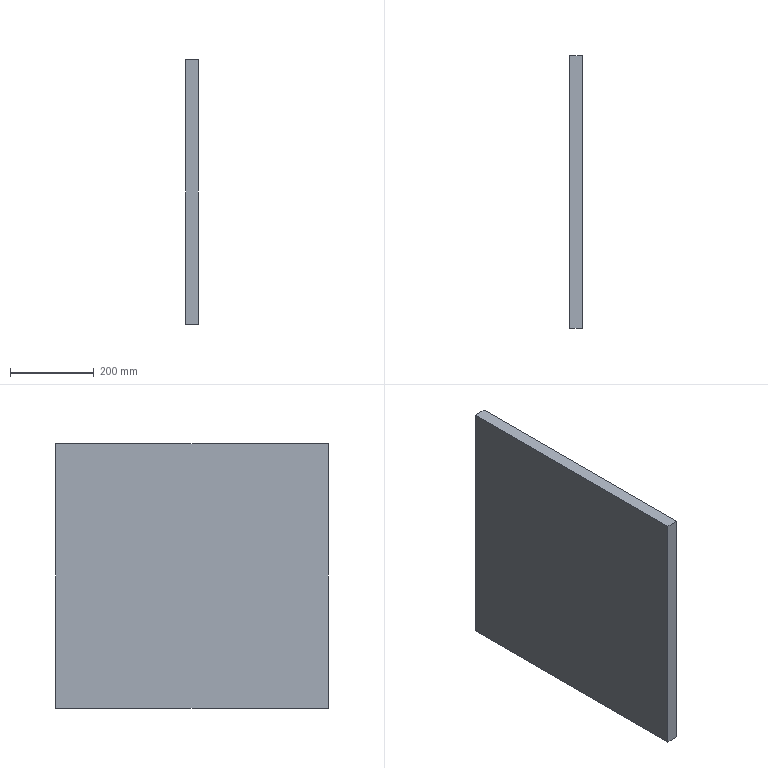Component | SolidWorks | ElectromagneticBeamEndPlate-1 | 1 solid | 6 faces | box 30 x 650 x 630 mm | volume 12285000 mm3 | plane 6 | material Plain Carbon Steel
STEP:
#1=COLOUR_RGB('',0.7922,0.8196,0.9333);
#2=FILL_AREA_STYLE_COLOUR('',#1);
#3=FILL_AREA_STYLE('',(#2));
#4=SURFACE_STYLE_FILL_AREA(#3);
#5=SURFACE_SIDE_STYLE('',(#4));
#6=SURFACE_STYLE_USAGE(.BOTH.,#5);
#7=PRESENTATION_STYLE_ASSIGNMENT((#6));
#8=CARTESIAN_POINT('',(-260.058,114.635,239.136));
#9=VERTEX_POINT('',#8);
#10=CARTESIAN_POINT('',(-260.058,114.635,263.939));
#11=VERTEX_POINT('',#10);
#12=CARTESIAN_POINT('',(-260.058,114.635,239.136));
#13=DIRECTION('',(-0.,0.,1.));
#14=VECTOR('',#13,39.37);
#15=LINE('',#12,#14);
#16=EDGE_CURVE('',#9,#11,#15,.T.);
#17=ORIENTED_EDGE('',*,*,#16,.F.);
#18=CARTESIAN_POINT('',(-258.877,114.635,239.136));
#19=VERTEX_POINT('',#18);
#20=CARTESIAN_POINT('',(-258.877,114.635,239.136));
#21=DIRECTION('',(-1.,-0.,0.));
#22=VECTOR('',#21,39.37);
#23=LINE('',#20,#22);
#24=EDGE_CURVE('',#19,#9,#23,.T.);
#25=ORIENTED_EDGE('',*,*,#24,.F.);
#26=CARTESIAN_POINT('',(-258.877,114.635,263.939));
#27=VERTEX_POINT('',#26);
#28=CARTESIAN_POINT('',(-258.877,114.635,239.136));
#29=DIRECTION('',(-0.,0.,1.));
#30=VECTOR('',#29,39.37);
#31=LINE('',#28,#30);
#32=EDGE_CURVE('',#19,#27,#31,.T.);
#33=ORIENTED_EDGE('',*,*,#32,.T.);
#34=CARTESIAN_POINT('',(-258.877,114.635,263.939));
#35=DIRECTION('',(-1.,-0.,0.));
#36=VECTOR('',#35,39.37);
#37=LINE('',#34,#36);
#38=EDGE_CURVE('',#27,#11,#37,.T.);
#39=ORIENTED_EDGE('',*,*,#38,.T.);
#40=EDGE_LOOP('',(#17,#25,#33,#39));
#41=FACE_OUTER_BOUND('',#40,.T.);
#42=CARTESIAN_POINT('',(-258.877,114.635,239.136));
#43=DIRECTION('',(0.,-1.,0.));
#44=DIRECTION('',(-0.,0.,1.));
#45=AXIS2_PLACEMENT_3D('',#42,#43,#44);
#46=PLANE('',#45);
#47=ADVANCED_FACE('',(#41),#46,.T.);
#48=CARTESIAN_POINT('',(-260.058,140.226,239.136));
#49=VERTEX_POINT('',#48);
#50=CARTESIAN_POINT('',(-260.058,114.635,239.136));
#51=DIRECTION('',(0.,-1.,0.));
#52=VECTOR('',#51,39.37);
#53=LINE('',#50,#52);
#54=EDGE_CURVE('',#49,#9,#53,.T.);
#55=ORIENTED_EDGE('',*,*,#54,.F.);
#56=CARTESIAN_POINT('',(-258.877,140.226,239.136));
#57=VERTEX_POINT('',#56);
#58=CARTESIAN_POINT('',(-258.877,140.226,239.136));
#59=DIRECTION('',(-1.,-0.,0.));
#60=VECTOR('',#59,39.37);
#61=LINE('',#58,#60);
#62=EDGE_CURVE('',#57,#49,#61,.T.);
#63=ORIENTED_EDGE('',*,*,#62,.F.);
#64=CARTESIAN_POINT('',(-258.877,114.635,239.136));
#65=DIRECTION('',(0.,-1.,0.));
#66=VECTOR('',#65,39.37);
#67=LINE('',#64,#66);
#68=EDGE_CURVE('',#57,#19,#67,.T.);
#69=ORIENTED_EDGE('',*,*,#68,.T.);
#70=ORIENTED_EDGE('',*,*,#24,.T.);
#71=EDGE_LOOP('',(#55,#63,#69,#70));
#72=FACE_OUTER_BOUND('',#71,.T.);
#73=CARTESIAN_POINT('',(-258.877,114.635,239.136));
#74=DIRECTION('',(0.,0.,-1.));
#75=DIRECTION('',(0.,-1.,0.));
#76=AXIS2_PLACEMENT_3D('',#73,#74,#75);
#77=PLANE('',#76);
#78=ADVANCED_FACE('',(#72),#77,.T.);
#79=CARTESIAN_POINT('',(-260.058,140.226,263.939));
#80=VERTEX_POINT('',#79);
#81=CARTESIAN_POINT('',(-260.058,140.226,239.136));
#82=DIRECTION('',(0.,-0.,-1.));
#83=VECTOR('',#82,39.37);
#84=LINE('',#81,#83);
#85=EDGE_CURVE('',#80,#49,#84,.T.);
#86=ORIENTED_EDGE('',*,*,#85,.F.);
#87=CARTESIAN_POINT('',(-258.877,140.226,263.939));
#88=VERTEX_POINT('',#87);
#89=CARTESIAN_POINT('',(-258.877,140.226,263.939));
#90=DIRECTION('',(-1.,-0.,0.));
#91=VECTOR('',#90,39.37);
#92=LINE('',#89,#91);
#93=EDGE_CURVE('',#88,#80,#92,.T.);
#94=ORIENTED_EDGE('',*,*,#93,.F.);
#95=CARTESIAN_POINT('',(-258.877,140.226,239.136));
#96=DIRECTION('',(0.,-0.,-1.));
#97=VECTOR('',#96,39.37);
#98=LINE('',#95,#97);
#99=EDGE_CURVE('',#88,#57,#98,.T.);
#100=ORIENTED_EDGE('',*,*,#99,.T.);
#101=ORIENTED_EDGE('',*,*,#62,.T.);
#102=EDGE_LOOP('',(#86,#94,#100,#101));
#103=FACE_OUTER_BOUND('',#102,.T.);
#104=CARTESIAN_POINT('',(-258.877,140.226,239.136));
#105=DIRECTION('',(-0.,1.,-0.));
#106=DIRECTION('',(0.,-0.,-1.));
#107=AXIS2_PLACEMENT_3D('',#104,#105,#106);
#108=PLANE('',#107);
#109=ADVANCED_FACE('',(#103),#108,.T.);
#110=CARTESIAN_POINT('',(-260.058,114.635,263.939));
#111=DIRECTION('',(-0.,1.,0.));
#112=VECTOR('',#111,39.37);
#113=LINE('',#110,#112);
#114=EDGE_CURVE('',#11,#80,#113,.T.);
#115=ORIENTED_EDGE('',*,*,#114,.F.);
#116=ORIENTED_EDGE('',*,*,#38,.F.);
#117=CARTESIAN_POINT('',(-258.877,114.635,263.939));
#118=DIRECTION('',(-0.,1.,0.));
#119=VECTOR('',#118,39.37);
#120=LINE('',#117,#119);
#121=EDGE_CURVE('',#27,#88,#120,.T.);
#122=ORIENTED_EDGE('',*,*,#121,.T.);
#123=ORIENTED_EDGE('',*,*,#93,.T.);
#124=EDGE_LOOP('',(#115,#116,#122,#123));
#125=FACE_OUTER_BOUND('',#124,.T.);
#126=CARTESIAN_POINT('',(-258.877,114.635,263.939));
#127=DIRECTION('',(0.,0.,1.));
#128=DIRECTION('',(-0.,1.,0.));
#129=AXIS2_PLACEMENT_3D('',#126,#127,#128);
#130=PLANE('',#129);
#131=ADVANCED_FACE('',(#125),#130,.T.);
#132=ORIENTED_EDGE('',*,*,#32,.F.);
#133=ORIENTED_EDGE('',*,*,#68,.F.);
#134=ORIENTED_EDGE('',*,*,#99,.F.);
#135=ORIENTED_EDGE('',*,*,#121,.F.);
#136=EDGE_LOOP('',(#132,#133,#134,#135));
#137=FACE_OUTER_BOUND('',#136,.T.);
#138=CARTESIAN_POINT('',(-258.877,114.635,239.136));
#139=DIRECTION('',(-1.,-0.,0.));
#140=DIRECTION('',(0.,0.,1.));
#141=AXIS2_PLACEMENT_3D('',#138,#139,#140);
#142=PLANE('',#141);
#143=ADVANCED_FACE('',(#137),#142,.F.);
#144=ORIENTED_EDGE('',*,*,#16,.T.);
#145=ORIENTED_EDGE('',*,*,#114,.T.);
#146=ORIENTED_EDGE('',*,*,#85,.T.);
#147=ORIENTED_EDGE('',*,*,#54,.T.);
#148=EDGE_LOOP('',(#144,#145,#146,#147));
#149=FACE_OUTER_BOUND('',#148,.T.);
#150=CARTESIAN_POINT('',(-260.058,114.635,239.136));
#151=DIRECTION('',(-1.,-0.,0.));
#152=DIRECTION('',(0.,0.,1.));
#153=AXIS2_PLACEMENT_3D('',#150,#151,#152);
#154=PLANE('',#153);
#155=ADVANCED_FACE('',(#149),#154,.T.);
#156=CLOSED_SHELL('',(#47,#78,#109,#131,#143,#155));
#157=MANIFOLD_SOLID_BREP('',#156);
#158=STYLED_ITEM('',(#7),#157);
#159=(LENGTH_UNIT()NAMED_UNIT(*)SI_UNIT($,.METRE.));
#160=LENGTH_MEASURE_WITH_UNIT(LENGTH_MEASURE(0.0254),#159);
#161=DIMENSIONAL_EXPONENTS(1.,0.,0.,0.,0.,0.,0.);
#162=(CONVERSION_BASED_UNIT('',#160)LENGTH_UNIT()NAMED_UNIT(#161));
#163=UNCERTAINTY_MEASURE_WITH_UNIT(LENGTH_MEASURE(0.00001),#162,'','');
#164=(NAMED_UNIT(*)PLANE_ANGLE_UNIT()SI_UNIT($,.RADIAN.));
#165=(NAMED_UNIT(*)SI_UNIT($,.STERADIAN.)SOLID_ANGLE_UNIT());
#166=(GEOMETRIC_REPRESENTATION_CONTEXT(3)GLOBAL_UNCERTAINTY_ASSIGNED_CONTEXT((#163))GLOBAL_UNIT_ASSIGNED_CONTEXT((#162,#164,#165))REPRESENTATION_CONTEXT('',''));
#167=MECHANICAL_DESIGN_GEOMETRIC_PRESENTATION_REPRESENTATION('',(#158),#166);
#168=PRESENTATION_LAYER_ASSIGNMENT('','',(#158));
#169=CARTESIAN_POINT('',(0.,0.,0.));
#170=DIRECTION('',(0.,0.,1.));
#171=DIRECTION('',(1.,0.,0.));
#172=AXIS2_PLACEMENT_3D('',#169,#170,#171);
#173=(LENGTH_UNIT()NAMED_UNIT(*)SI_UNIT($,.METRE.));
#174=LENGTH_MEASURE_WITH_UNIT(LENGTH_MEASURE(0.0254),#173);
#175=DIMENSIONAL_EXPONENTS(1.,0.,0.,0.,0.,0.,0.);
#176=(CONVERSION_BASED_UNIT('',#174)LENGTH_UNIT()NAMED_UNIT(#175));
#177=UNCERTAINTY_MEASURE_WITH_UNIT(LENGTH_MEASURE(0.00001),#176,'','');
#178=(NAMED_UNIT(*)PLANE_ANGLE_UNIT()SI_UNIT($,.RADIAN.));
#179=(NAMED_UNIT(*)SI_UNIT($,.STERADIAN.)SOLID_ANGLE_UNIT());
#180=(GEOMETRIC_REPRESENTATION_CONTEXT(3)GLOBAL_UNCERTAINTY_ASSIGNED_CONTEXT((#177))GLOBAL_UNIT_ASSIGNED_CONTEXT((#176,#178,#179))REPRESENTATION_CONTEXT('',''));
#181=ADVANCED_BREP_SHAPE_REPRESENTATION('',(#157,#172),#180);